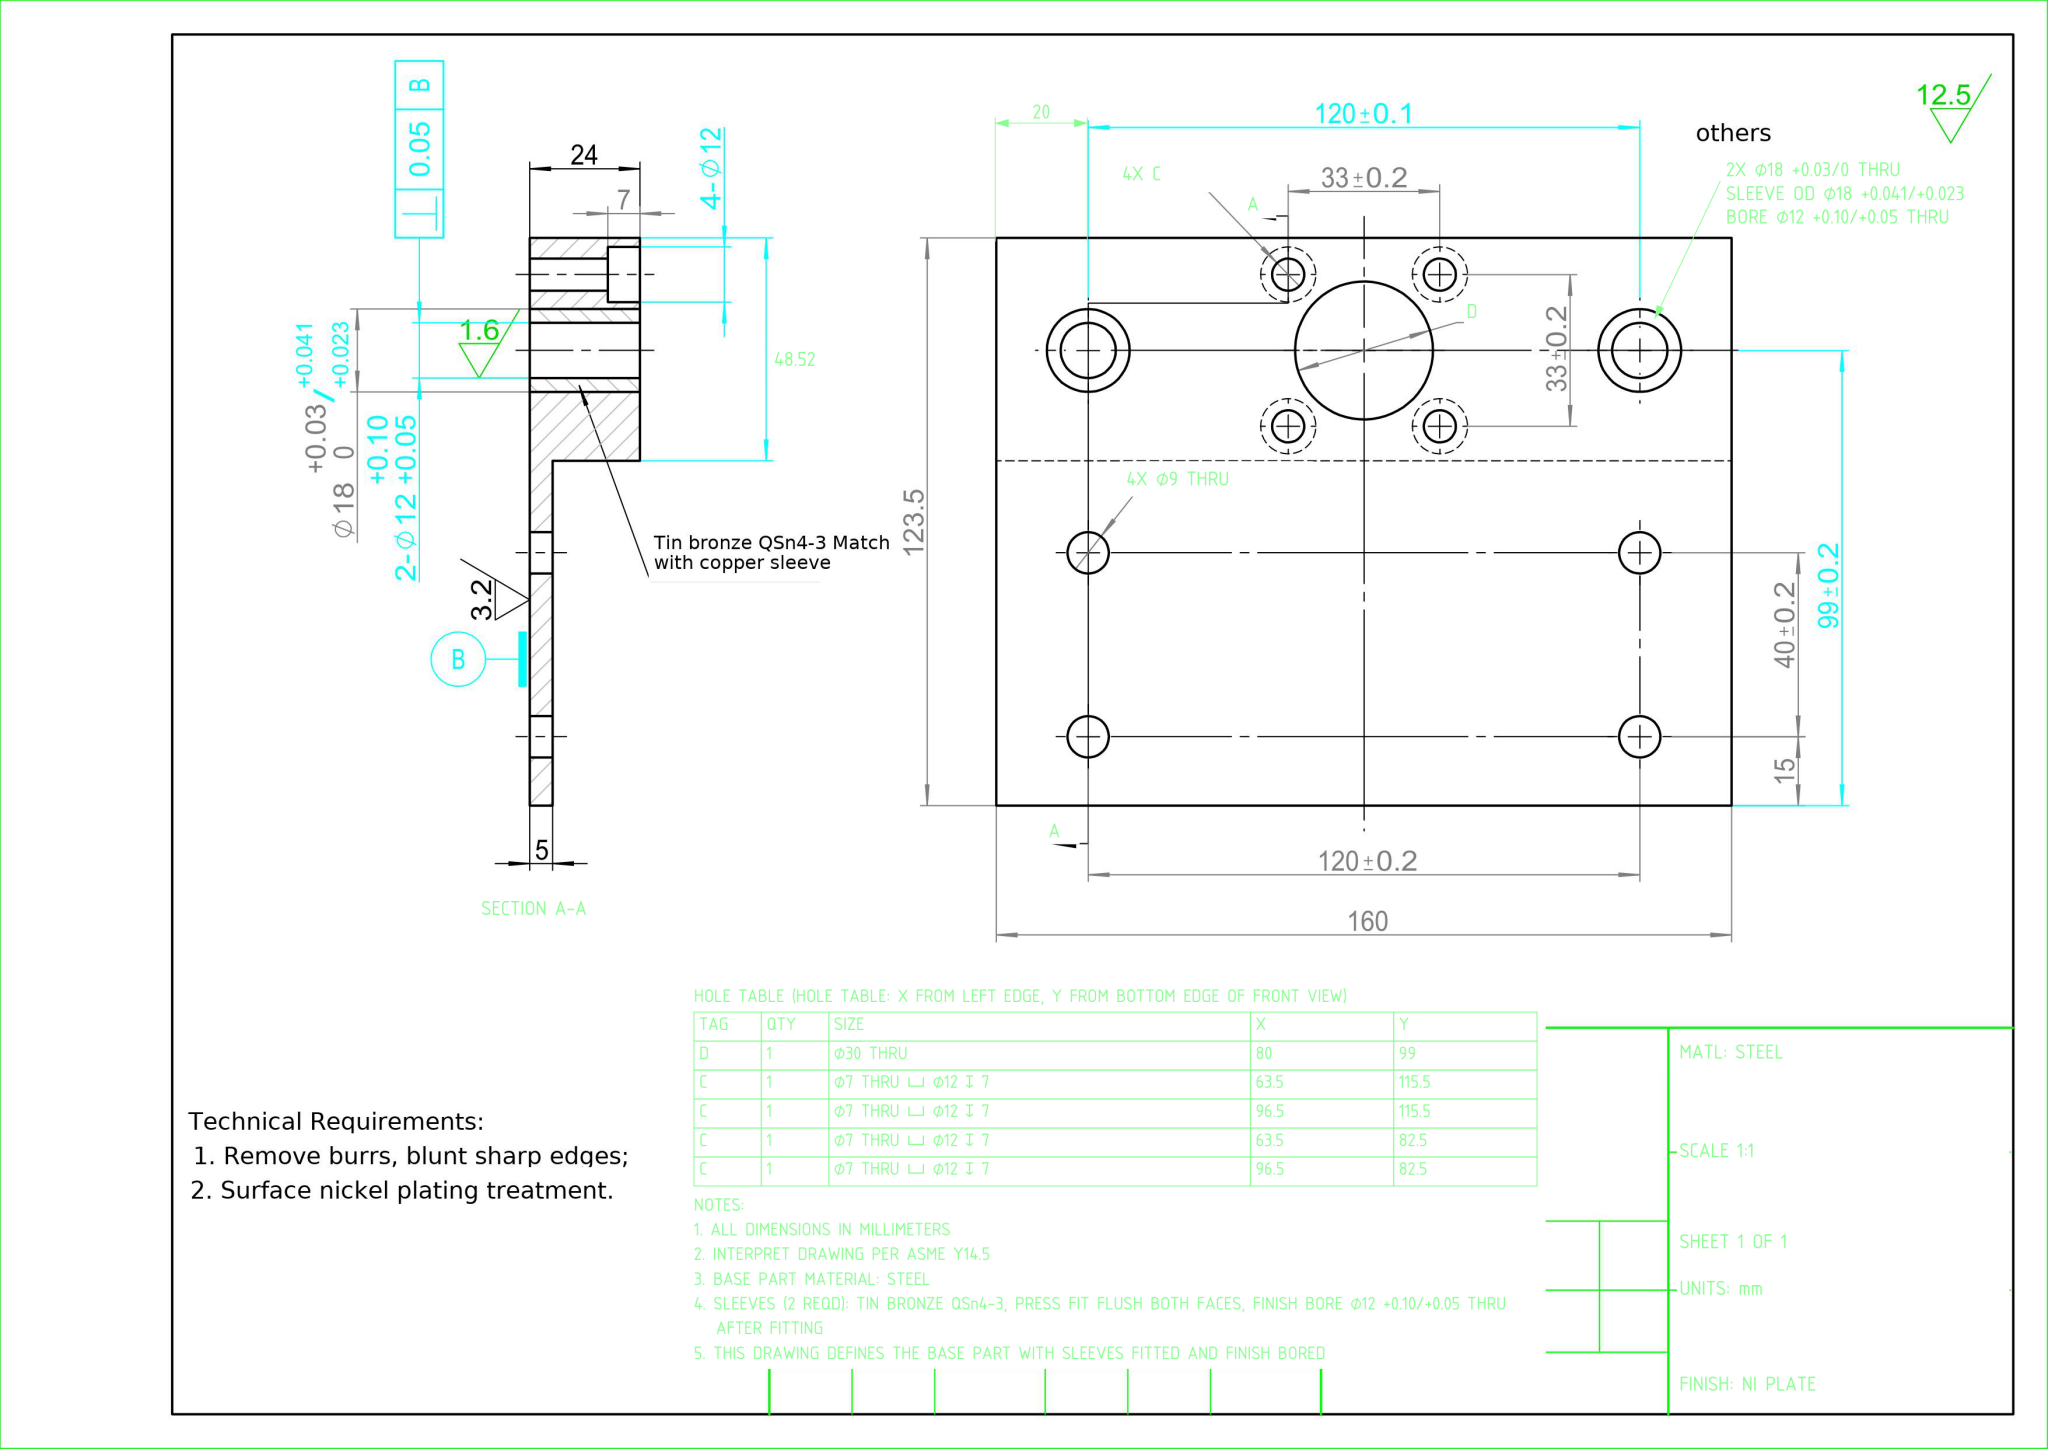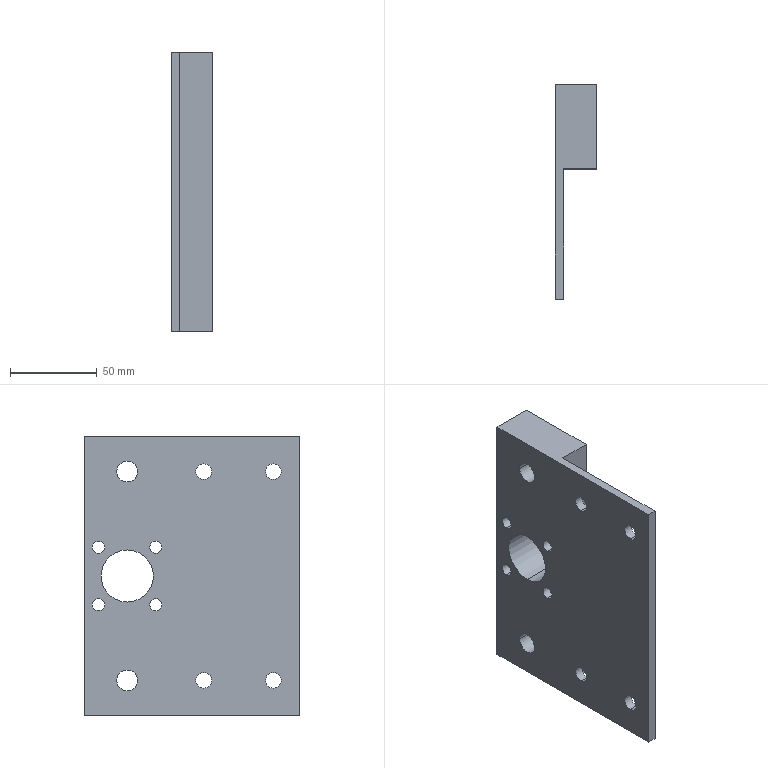Part | NX | mm | 1 solid | 42 faces | box 24 x 123.5 x 160 mm | volume 216852 mm3 | cylinder 30 | plane 12 | commonest cylinder face diameters 12 x12 7 x8 9 x8 30 x2